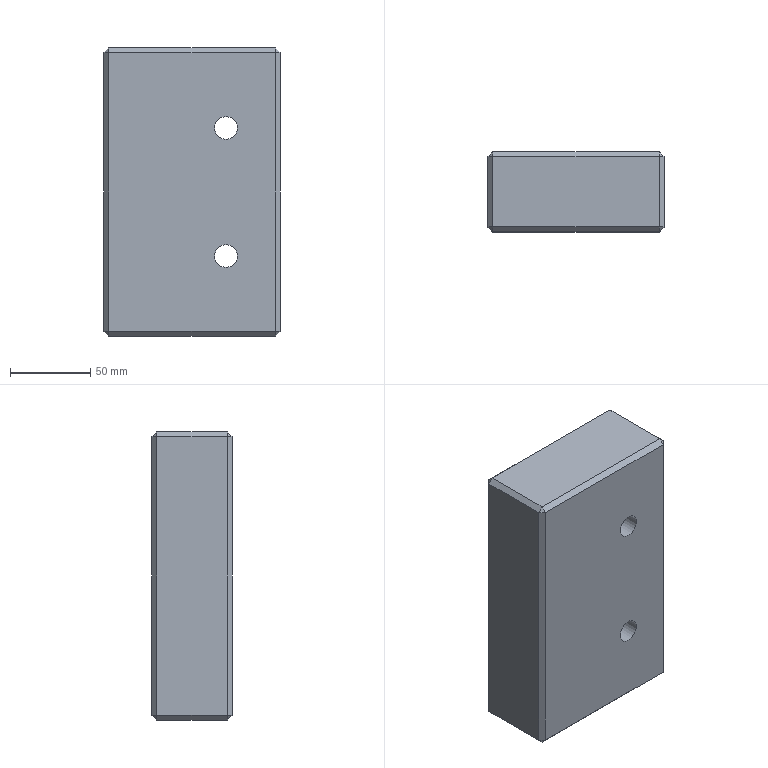Component | NX | SUPPORTING_PLATE_2 | 1 solid | 34 faces | volume 956802 mm3 | plane 28 | cylinder 4 | torus 2 | commonest cylinder face diameters 14.2 x2 25.9 x2